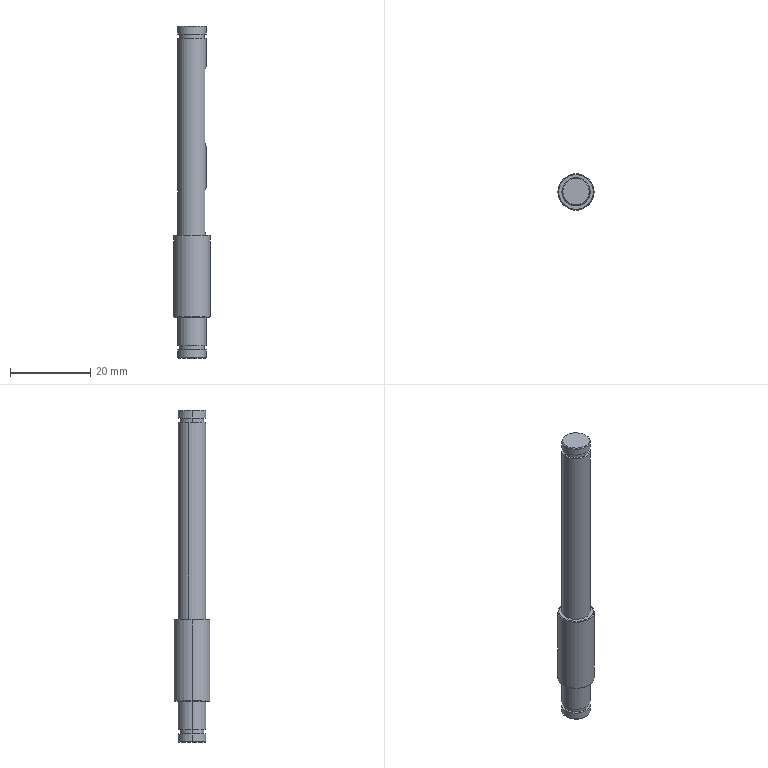CAM job | Mastercam | mm | 3 operations | part box 9 x 9 x 82.7
1. Contour (Ramp) | 2 - 2 平铣刀
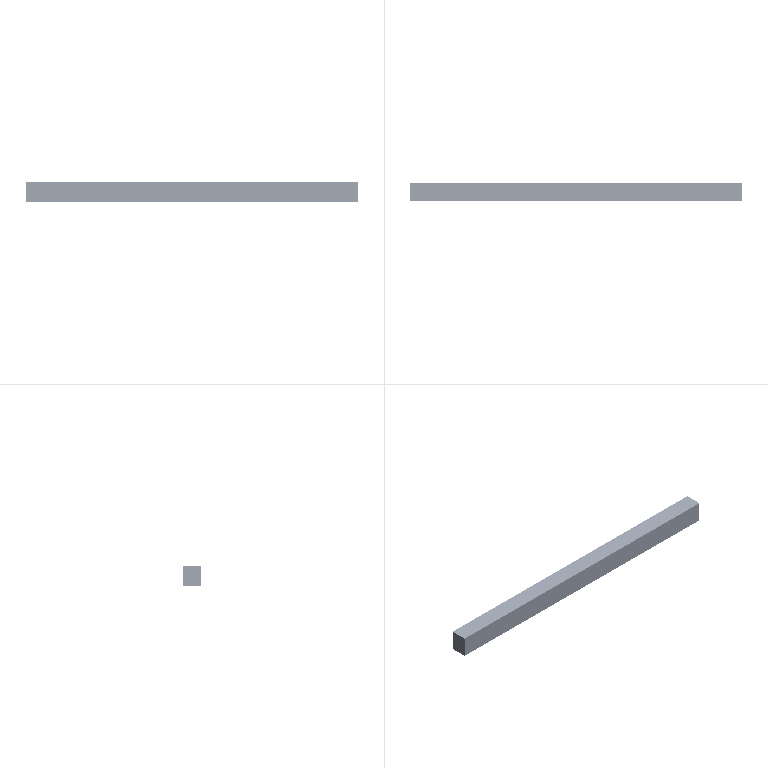2. Contour (Ramp) | 2 - 2 平铣刀
3. Deburr 5-axis | 1 - 2 球刀/圆鼻铣刀